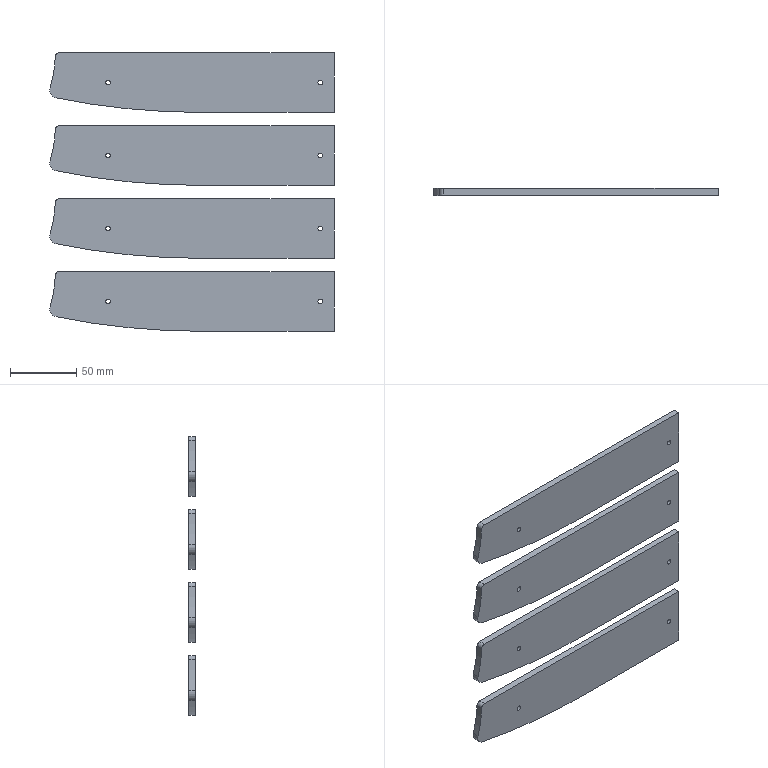CAM job | Mastercam | mm | 4 operations | part box 214.46 x 5 x 210
1. Contour (Ramp) | 3 - 3 平铣刀
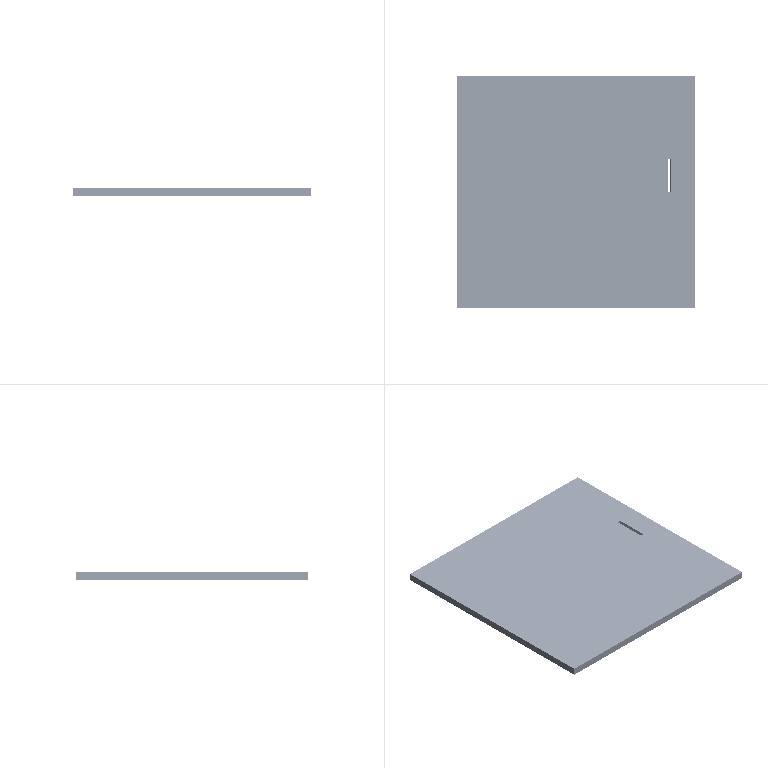2. Contour (2D) | 3 - 3 平铣刀
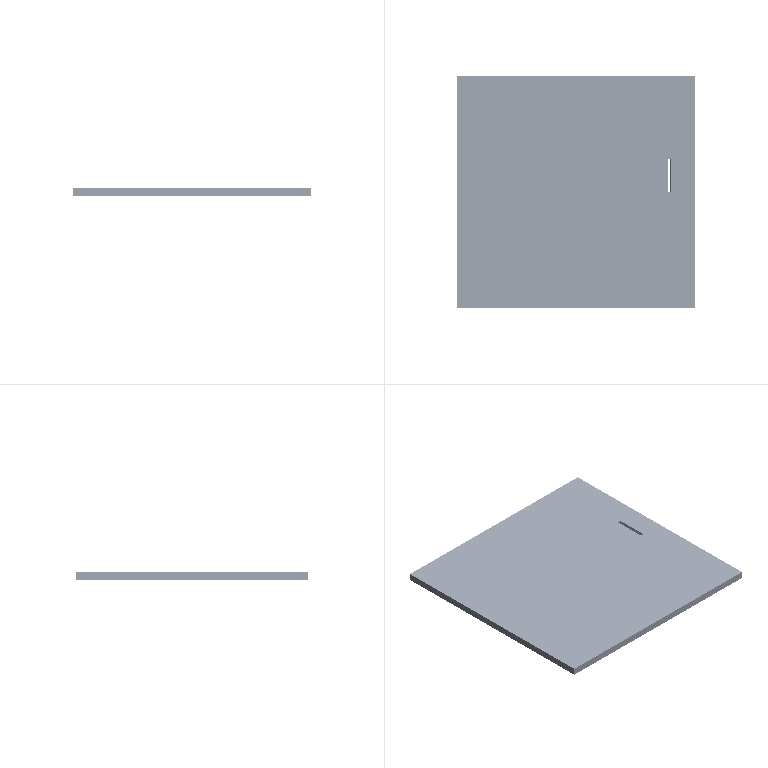3. Drill/Counterbore | 7 - 4 倒角刀
4. Contour (2D chamfer) | 7 - 4 倒角刀